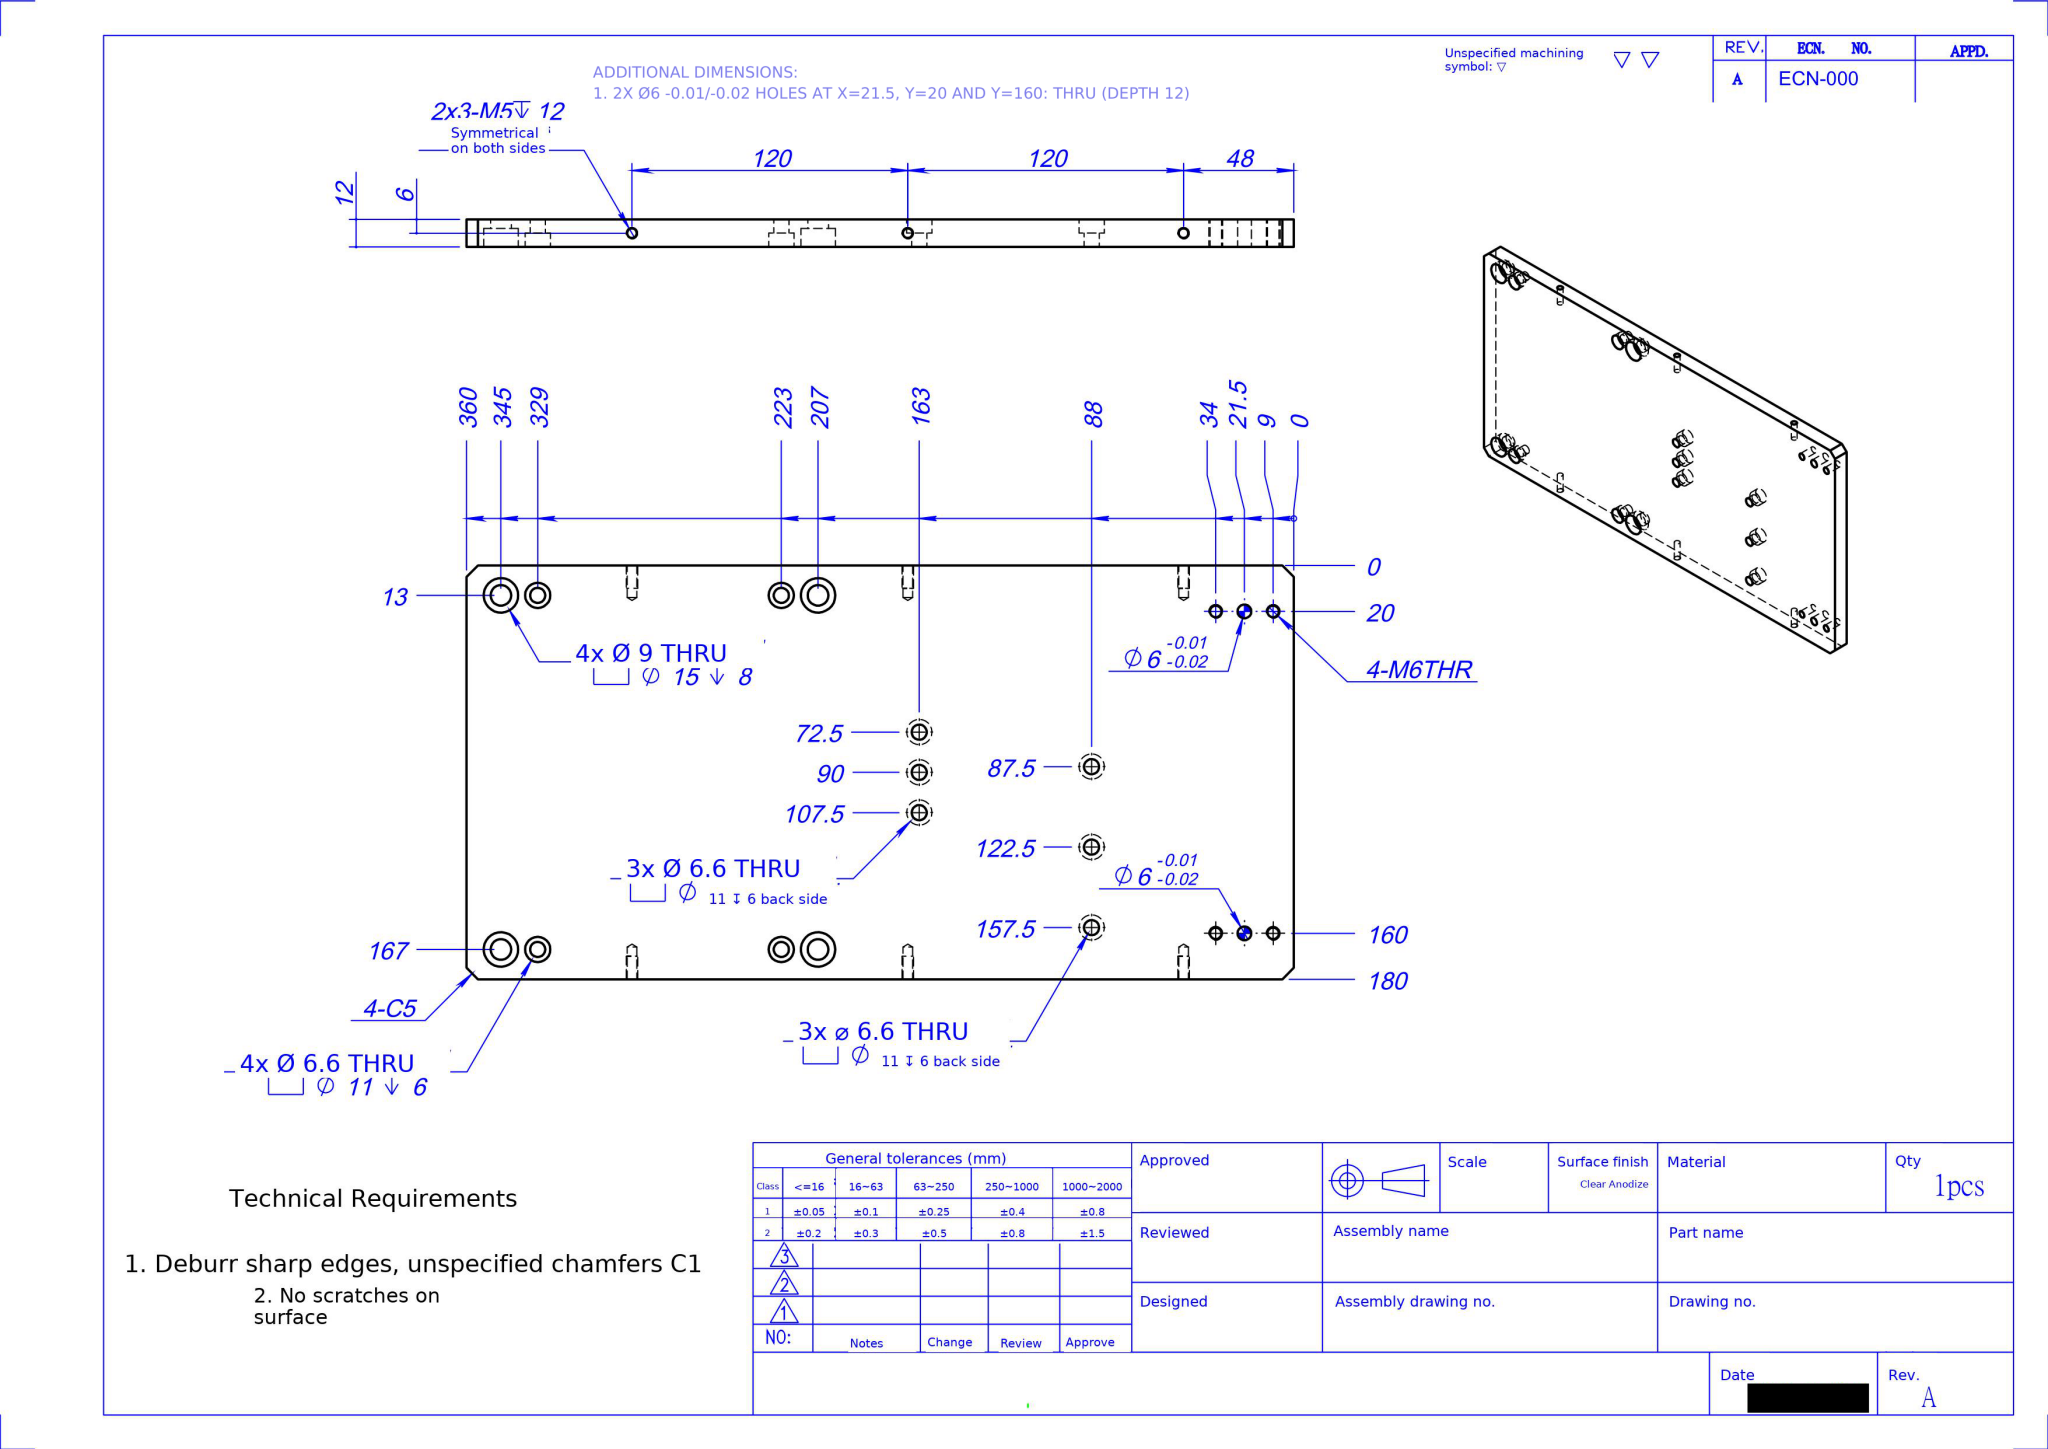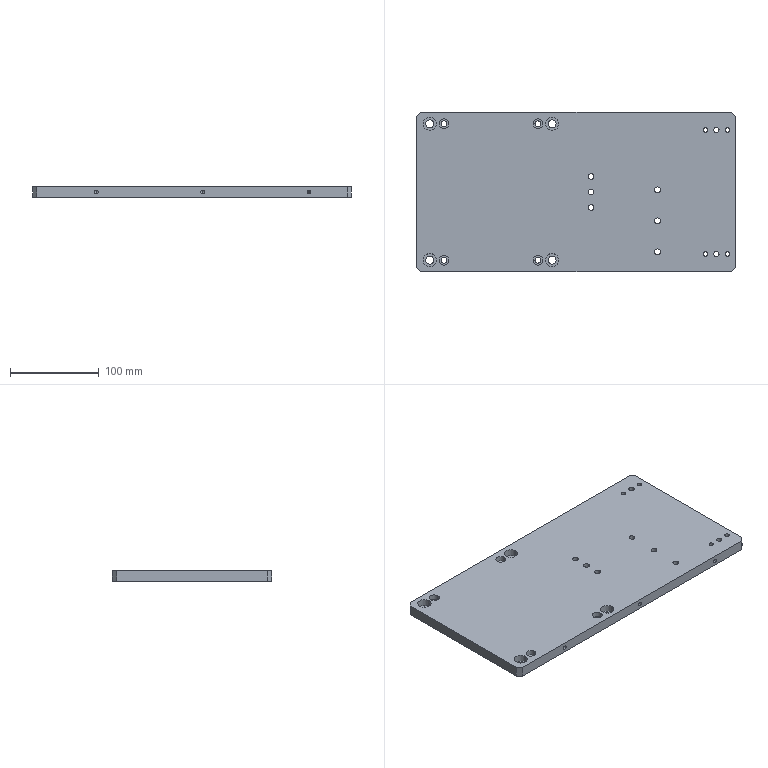Part | NX | mm | 1 solid | 116 faces | box 360 x 180 x 12 mm | volume 759753 mm3 | cylinder 80 | plane 24 | cone 12 | commonest cylinder face diameters 6.6 x20 11 x20 4.2 x12 5 x8 9 x8 15 x8 6 x4